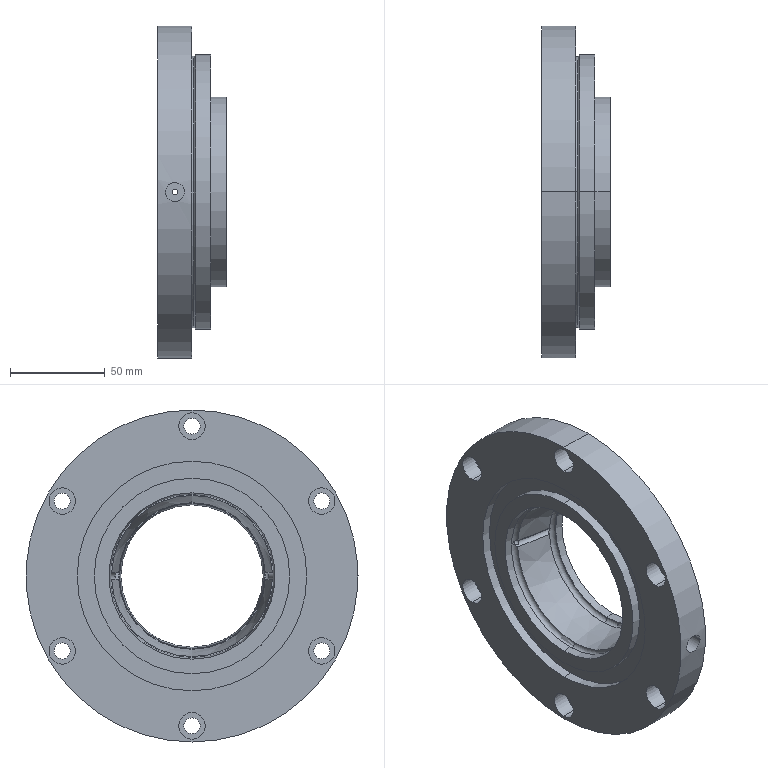Component | SolidWorks | 26TaperSleeve-1 | 1 solid | 78 faces | volume 438760 mm3 | cylinder 47 | plane 16 | cone 11 | torus 4 | commonest cylinder face diameters 14 x12 8.5 x12 3 x4 10 x4 4 x3 103 x2 121 x2 100 x2